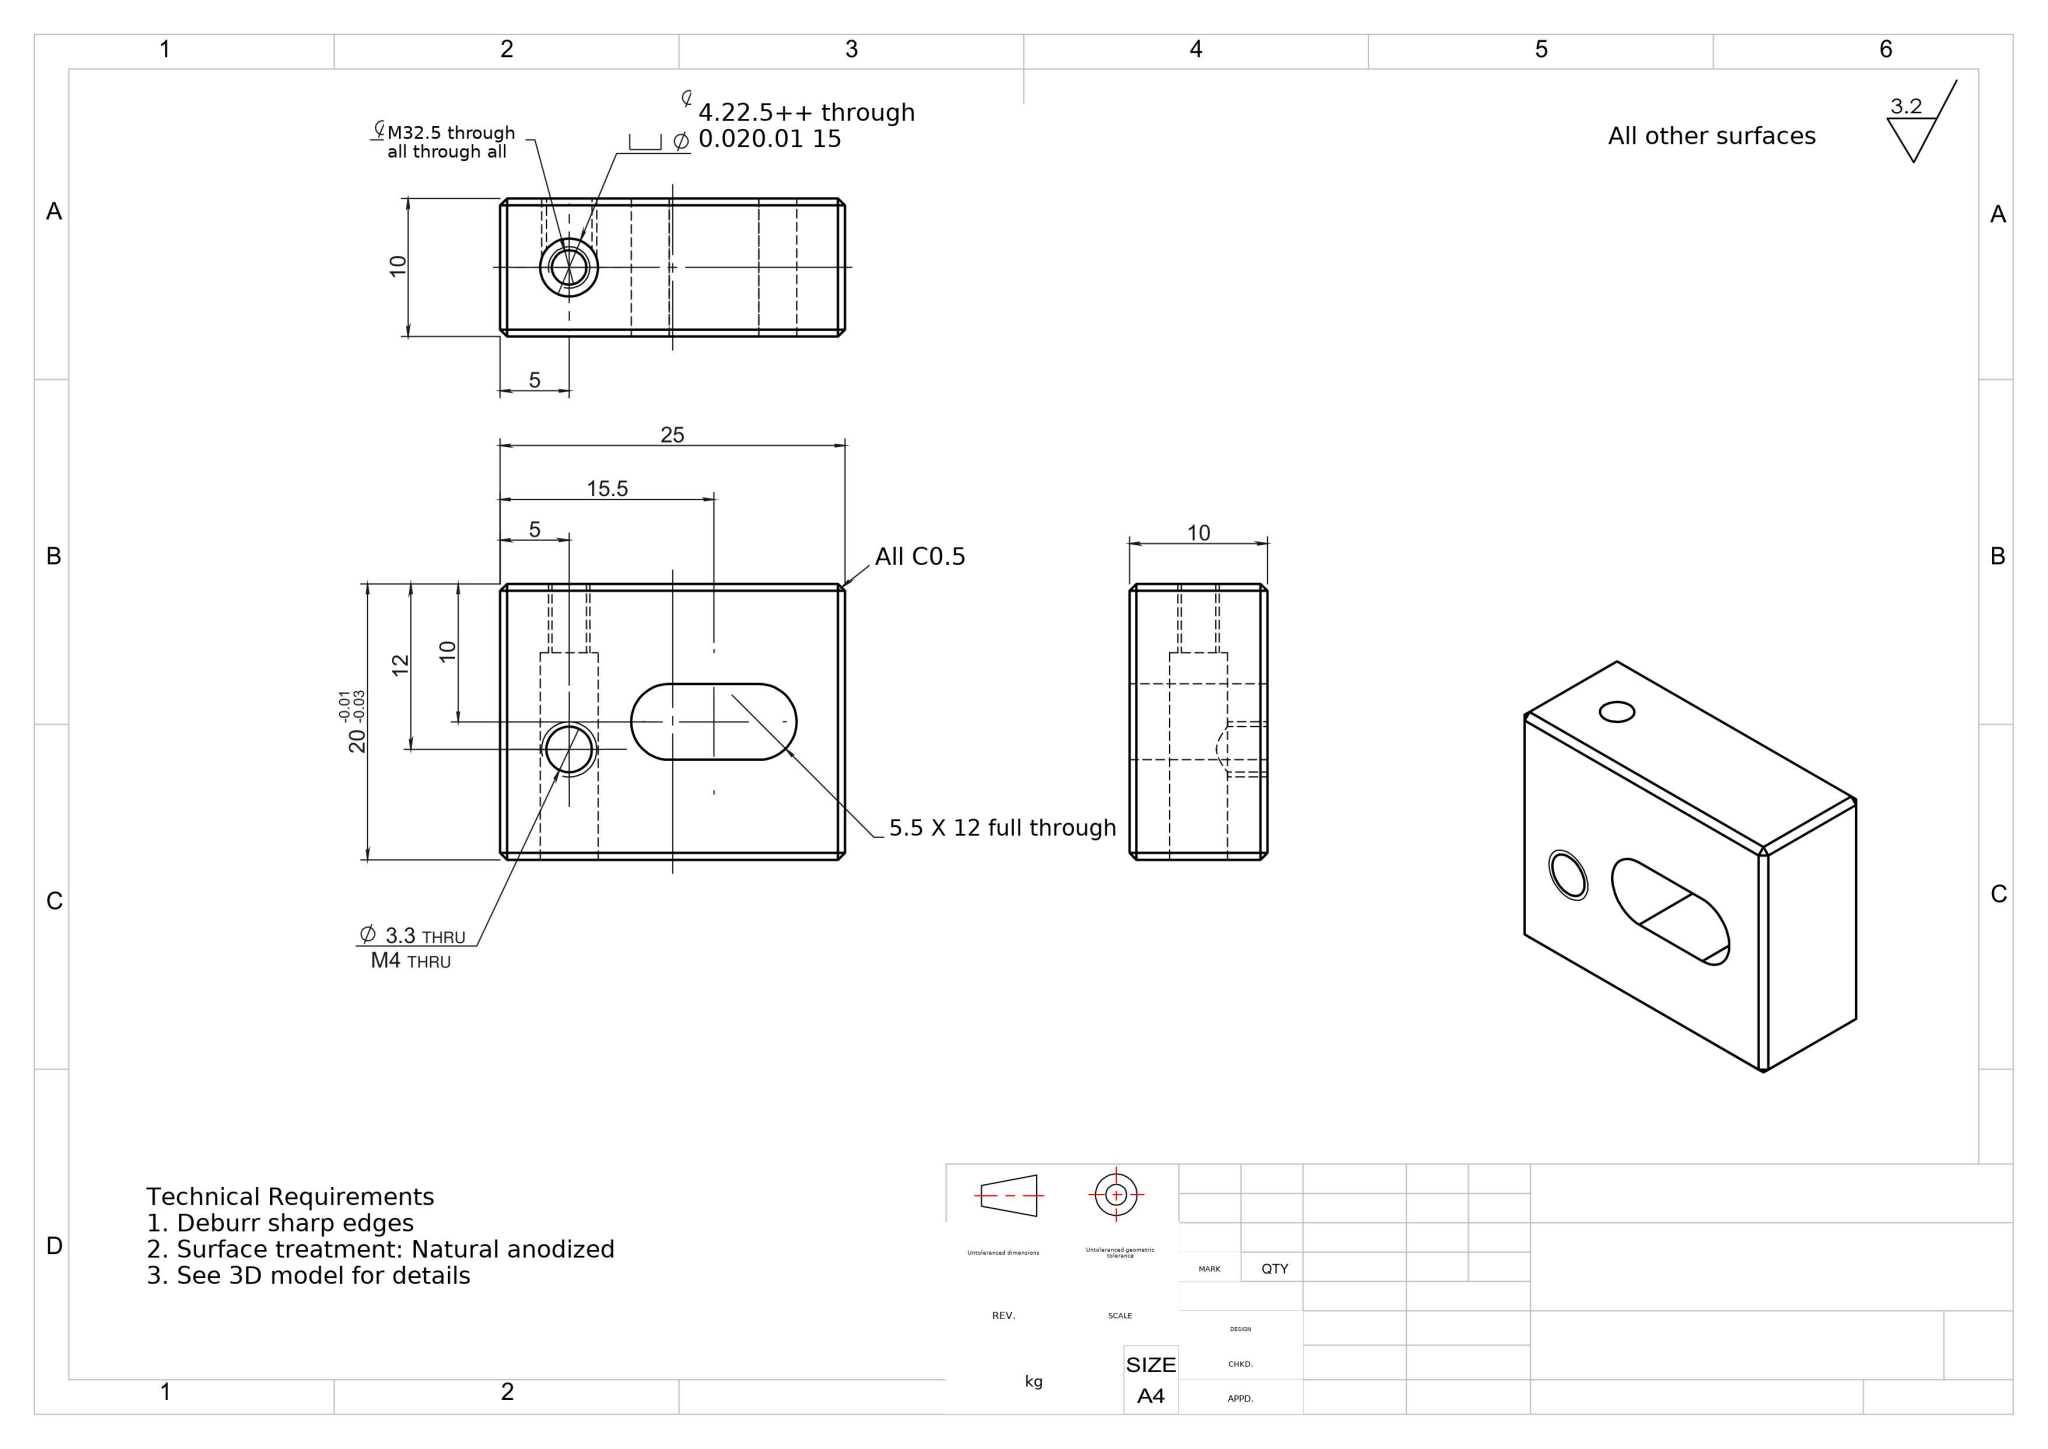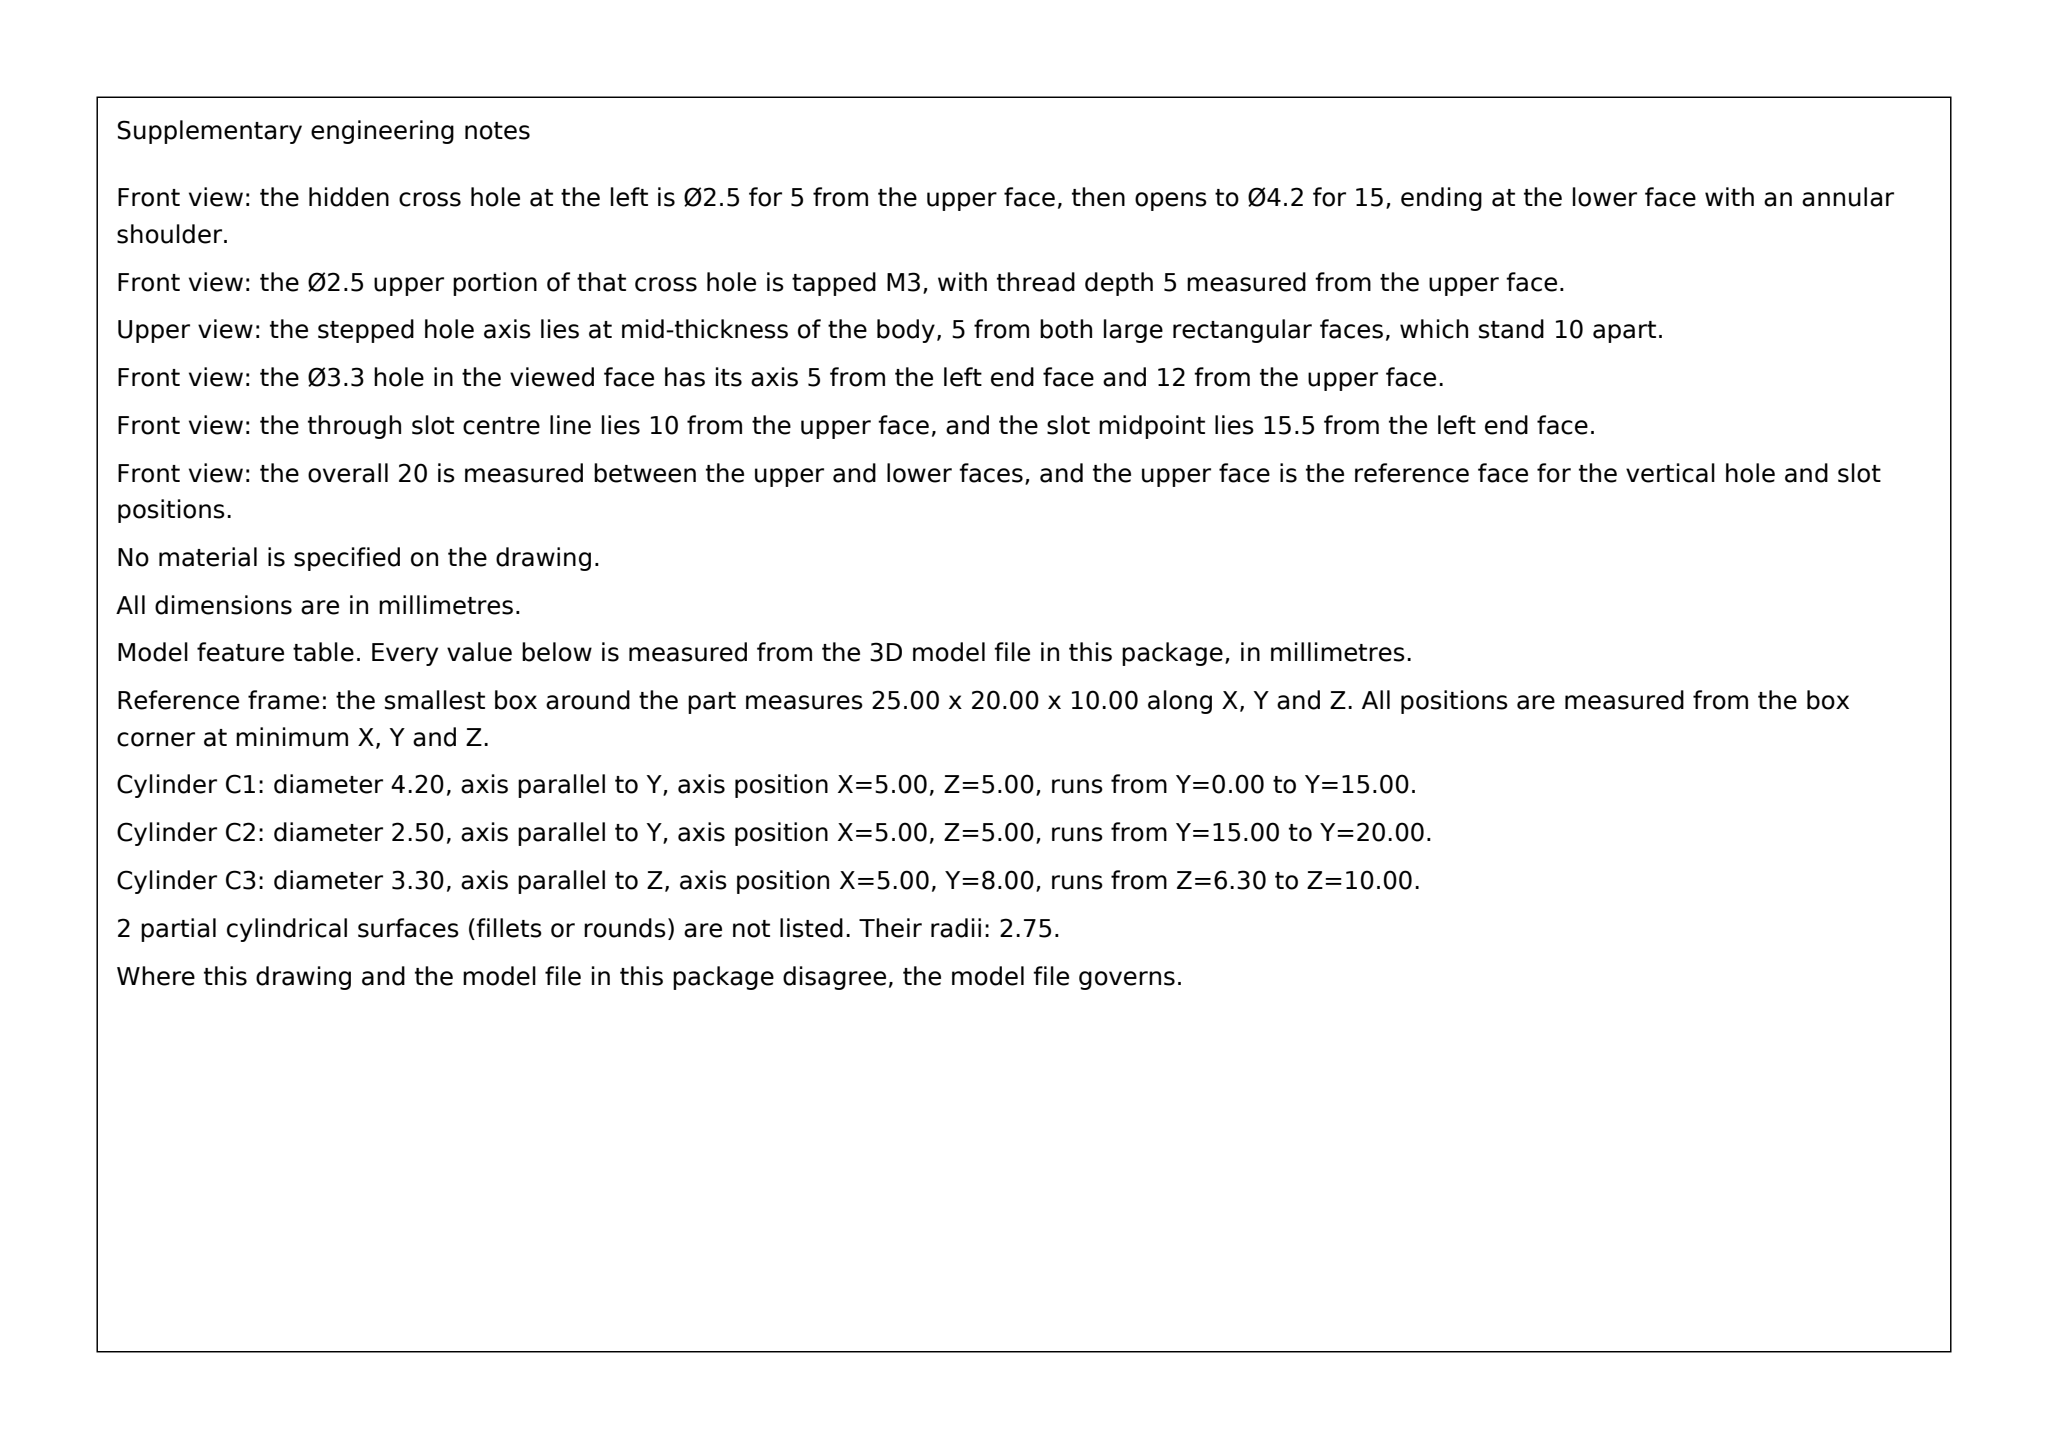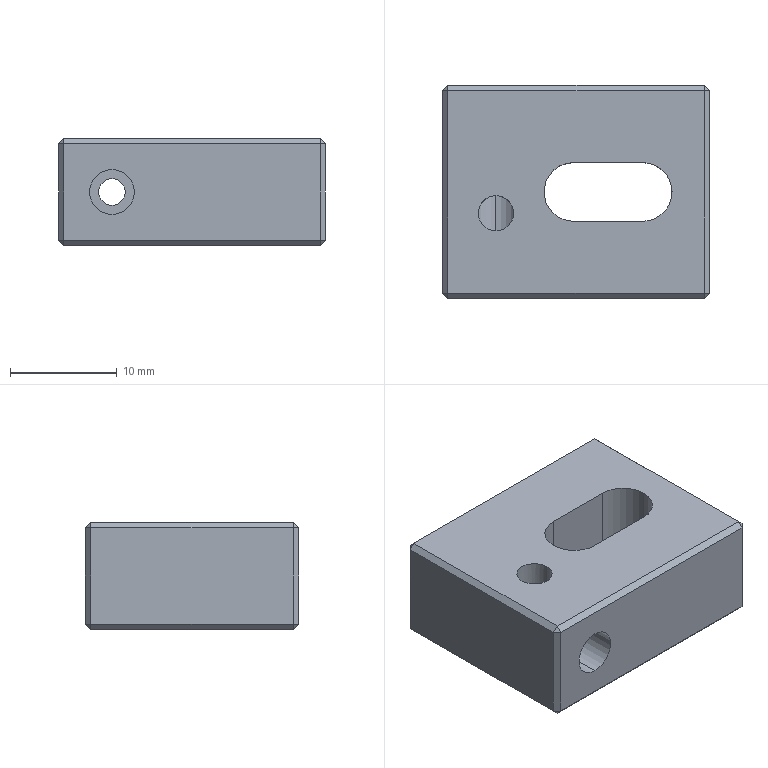Part | SolidWorks | mm | 1 solid | 38 faces | box 25 x 20 x 10 mm | volume 4119 mm3 | plane 29 | cylinder 9 | commonest cylinder face diameters 5.5 x3 3.3 x2 2.5 x2 4.2 x2
Drawing notes:
M3 TAPPED HOLE, TAP DRILL Ø2.5, 5 DEEP FROM TOP FACE (Y=20); AXIS 5 FROM LEFT END (X=5) AND AT MID-THICKNESS (Z=5) | from the solid: cylinder [2.5, axis y, pos (x=5.0, z=5.0), length 5.0] with y planes at 15.0 and 20.0
Ø4.2 CLEARANCE HOLE, 15 DEEP FROM BOTTOM FACE (Y=0), COAXIAL WITH M3; X=5, Z=5 | from the solid: cylinder [4.2, axis y, pos (x=5.0, z=5.0), length 15.0] with y planes at 0.0 and 15.0
ALL DIMENSIONS IN MILLIMETERS; OVERALL SIZE 25 x 20 x 10 | from the solid: STEP units mm, bbox_xyz [25.0, 20.0, 10.0]